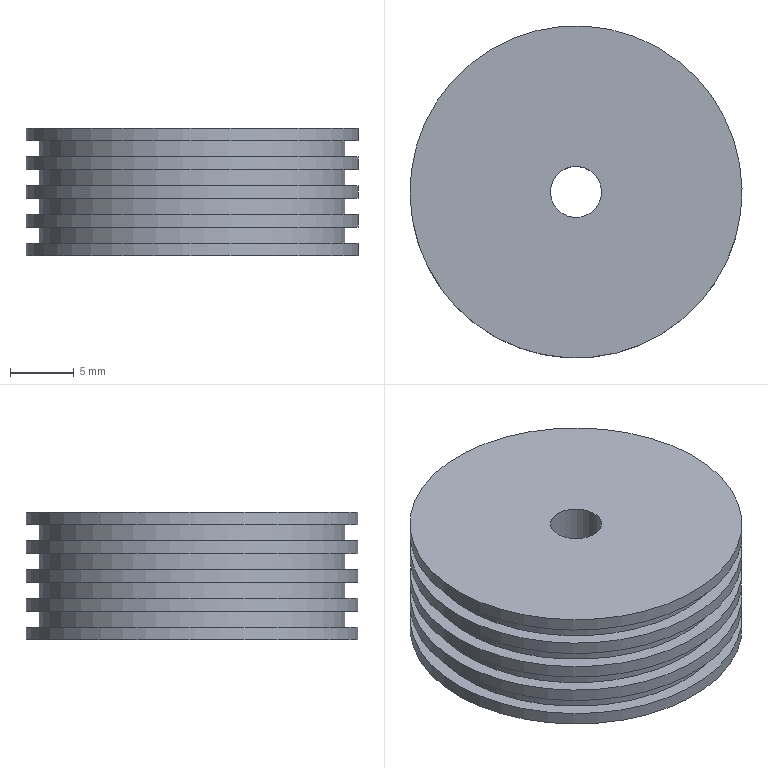Component | NX | 18A__27_2 | 1 solid | 20 faces | box 26 x 26 x 10 mm | volume 4791 mm3 | plane 10 | cylinder 10 | commonest cylinder face diameters 26 x5 24 x4 4 x1
STEP:
#1=CARTESIAN_POINT('',(0.,0.,0.));
#2=DIRECTION('',(0.,0.,1.));
#3=DIRECTION('',(1.,0.,0.));
#4=AXIS2_PLACEMENT_3D('',#1,#2,#3);
#5=CARTESIAN_POINT('',(16.256,111.456,213.535));
#6=VERTEX_POINT('',#5);
#7=CARTESIAN_POINT('',(17.022,109.608,213.535));
#8=DIRECTION('',(0.,0.,1.));
#9=DIRECTION('',(-0.383,0.9237,0.));
#10=AXIS2_PLACEMENT_3D('',#7,#8,#9);
#11=CIRCLE('',#10,2.);
#12=CARTESIAN_POINT('',(22.002,97.6,213.535));
#13=DIRECTION('',(0.,0.,-1.));
#14=DIRECTION('',(0.383,-0.9237,0.));
#15=AXIS2_PLACEMENT_3D('',#12,#13,#14);
#16=PLANE('',#15);
#17=CARTESIAN_POINT('',(-15.,0.));
#18=CARTESIAN_POINT('',(-15.,3.464));
#19=CARTESIAN_POINT('',(-12.,1.732));
#20=CARTESIAN_POINT('',(-9.,0.));
#21=CARTESIAN_POINT('',(-12.,-1.732));
#22=CARTESIAN_POINT('',(-15.,-3.464));
#23=CARTESIAN_POINT('',(-15.,0.));
#24=(BOUNDED_CURVE()B_SPLINE_CURVE(2,(#17,#18,#19,#20,#21,#22,#23),.UNSPECIFIED.,.T.,.F.)B_SPLINE_CURVE_WITH_KNOTS((1,2,2,2,2,1),(-2.094,0.,2.094,4.189,6.283,8.378),.UNSPECIFIED.)CURVE()GEOMETRIC_REPRESENTATION_ITEM()RATIONAL_B_SPLINE_CURVE((1.,0.5,1.,0.5,1.,0.5,1.))REPRESENTATION_ITEM(''));
#25=(GEOMETRIC_REPRESENTATION_CONTEXT(2)PARAMETRIC_REPRESENTATION_CONTEXT()REPRESENTATION_CONTEXT('',''));
#26=DEFINITIONAL_REPRESENTATION('',(#24),#25);
#27=PCURVE('',#16,#26);
#28=CARTESIAN_POINT('',(17.022,109.608,213.535));
#29=DIRECTION('',(0.,0.,1.));
#30=DIRECTION('',(-0.383,0.9237,0.));
#31=AXIS2_PLACEMENT_3D('',#28,#29,#30);
#32=CYLINDRICAL_SURFACE('',#31,2.);
#33=CARTESIAN_POINT('',(0.,0.));
#34=DIRECTION('',(1.,0.));
#35=VECTOR('',#34,1.);
#36=LINE('',#33,#35);
#37=(GEOMETRIC_REPRESENTATION_CONTEXT(2)PARAMETRIC_REPRESENTATION_CONTEXT()REPRESENTATION_CONTEXT('',''));
#38=DEFINITIONAL_REPRESENTATION('',(#36),#37);
#39=PCURVE('',#32,#38);
#40=SURFACE_CURVE('',#11,(#27,#39),.PCURVE_S1.);
#41=EDGE_CURVE('',#6,#6,#40,.T.);
#42=ORIENTED_EDGE('',*,*,#41,.T.);
#43=EDGE_LOOP('',(#42));
#44=FACE_BOUND('',#43,.T.);
#45=CARTESIAN_POINT('',(12.043,121.617,213.535));
#46=VERTEX_POINT('',#45);
#47=CARTESIAN_POINT('',(17.022,109.608,213.535));
#48=DIRECTION('',(0.,0.,1.));
#49=DIRECTION('',(-0.383,0.9237,0.));
#50=AXIS2_PLACEMENT_3D('',#47,#48,#49);
#51=CIRCLE('',#50,13.);
#52=CARTESIAN_POINT('',(-26.,0.));
#53=CARTESIAN_POINT('',(-26.,22.517));
#54=CARTESIAN_POINT('',(-6.5,11.258));
#55=CARTESIAN_POINT('',(13.,0.));
#56=CARTESIAN_POINT('',(-6.5,-11.258));
#57=CARTESIAN_POINT('',(-26.,-22.517));
#58=CARTESIAN_POINT('',(-26.,0.));
#59=(BOUNDED_CURVE()B_SPLINE_CURVE(2,(#52,#53,#54,#55,#56,#57,#58),.UNSPECIFIED.,.T.,.F.)B_SPLINE_CURVE_WITH_KNOTS((1,2,2,2,2,1),(-2.094,0.,2.094,4.189,6.283,8.378),.UNSPECIFIED.)CURVE()GEOMETRIC_REPRESENTATION_ITEM()RATIONAL_B_SPLINE_CURVE((1.,0.5,1.,0.5,1.,0.5,1.))REPRESENTATION_ITEM(''));
#60=(GEOMETRIC_REPRESENTATION_CONTEXT(2)PARAMETRIC_REPRESENTATION_CONTEXT()REPRESENTATION_CONTEXT('',''));
#61=DEFINITIONAL_REPRESENTATION('',(#59),#60);
#62=PCURVE('',#16,#61);
#63=CARTESIAN_POINT('',(17.022,109.608,213.535));
#64=DIRECTION('',(0.,0.,1.));
#65=DIRECTION('',(-0.383,0.9237,0.));
#66=AXIS2_PLACEMENT_3D('',#63,#64,#65);
#67=CYLINDRICAL_SURFACE('',#66,13.);
#68=CARTESIAN_POINT('',(0.,0.));
#69=DIRECTION('',(1.,0.));
#70=VECTOR('',#69,1.);
#71=LINE('',#68,#70);
#72=(GEOMETRIC_REPRESENTATION_CONTEXT(2)PARAMETRIC_REPRESENTATION_CONTEXT()REPRESENTATION_CONTEXT('',''));
#73=DEFINITIONAL_REPRESENTATION('',(#71),#72);
#74=PCURVE('',#67,#73);
#75=SURFACE_CURVE('',#51,(#62,#74),.PCURVE_S1.);
#76=EDGE_CURVE('',#46,#46,#75,.T.);
#77=ORIENTED_EDGE('',*,*,#76,.F.);
#78=EDGE_LOOP('',(#77));
#79=FACE_BOUND('',#78,.T.);
#80=ADVANCED_FACE('',(#44,#79),#16,.T.);
#81=CARTESIAN_POINT('',(16.256,111.456,223.535));
#82=VERTEX_POINT('',#81);
#83=CARTESIAN_POINT('',(17.022,109.608,223.535));
#84=DIRECTION('',(0.,0.,1.));
#85=DIRECTION('',(-0.383,0.9237,0.));
#86=AXIS2_PLACEMENT_3D('',#83,#84,#85);
#87=CIRCLE('',#86,2.);
#88=CARTESIAN_POINT('',(0.,10.));
#89=DIRECTION('',(1.,0.));
#90=VECTOR('',#89,1.);
#91=LINE('',#88,#90);
#92=(GEOMETRIC_REPRESENTATION_CONTEXT(2)PARAMETRIC_REPRESENTATION_CONTEXT()REPRESENTATION_CONTEXT('',''));
#93=DEFINITIONAL_REPRESENTATION('',(#91),#92);
#94=PCURVE('',#32,#93);
#95=CARTESIAN_POINT('',(17.788,107.761,223.535));
#96=DIRECTION('',(0.,0.,1.));
#97=DIRECTION('',(-0.383,0.9237,0.));
#98=AXIS2_PLACEMENT_3D('',#95,#96,#97);
#99=PLANE('',#98);
#100=CARTESIAN_POINT('',(2.,0.));
#101=DIRECTION('',(1.,0.));
#102=AXIS2_PLACEMENT_2D('',#100,#101);
#103=CIRCLE('',#102,2.);
#104=(GEOMETRIC_REPRESENTATION_CONTEXT(2)PARAMETRIC_REPRESENTATION_CONTEXT()REPRESENTATION_CONTEXT('',''));
#105=DEFINITIONAL_REPRESENTATION('',(#103),#104);
#106=PCURVE('',#99,#105);
#107=SURFACE_CURVE('',#87,(#94,#106),.PCURVE_S1.);
#108=EDGE_CURVE('',#82,#82,#107,.T.);
#109=ORIENTED_EDGE('',*,*,#108,.F.);
#110=CARTESIAN_POINT('',(16.256,111.456,213.535));
#111=CARTESIAN_POINT('',(16.256,111.456,223.535));
#112=B_SPLINE_CURVE_WITH_KNOTS('',1,(#110,#111),.UNSPECIFIED.,.F.,.F.,(2,2),(0.,10.),.PIECEWISE_BEZIER_KNOTS.);
#113=CARTESIAN_POINT('',(0.,0.));
#114=DIRECTION('',(0.,1.));
#115=VECTOR('',#114,1.);
#116=LINE('',#113,#115);
#117=(GEOMETRIC_REPRESENTATION_CONTEXT(2)PARAMETRIC_REPRESENTATION_CONTEXT()REPRESENTATION_CONTEXT('',''));
#118=DEFINITIONAL_REPRESENTATION('',(#116),#117);
#119=PCURVE('',#32,#118);
#120=CARTESIAN_POINT('',(6.283,0.));
#121=DIRECTION('',(0.,1.));
#122=VECTOR('',#121,1.);
#123=LINE('',#120,#122);
#124=(GEOMETRIC_REPRESENTATION_CONTEXT(2)PARAMETRIC_REPRESENTATION_CONTEXT()REPRESENTATION_CONTEXT('',''));
#125=DEFINITIONAL_REPRESENTATION('',(#123),#124);
#126=PCURVE('',#32,#125);
#127=SEAM_CURVE('',#112,(#119,#126),.PCURVE_S1.);
#128=EDGE_CURVE('',#6,#82,#127,.T.);
#129=ORIENTED_EDGE('',*,*,#128,.F.);
#130=ORIENTED_EDGE('',*,*,#41,.T.);
#131=ORIENTED_EDGE('',*,*,#128,.T.);
#132=EDGE_LOOP('',(#109,#129,#130,#131));
#133=FACE_BOUND('',#132,.F.);
#134=ADVANCED_FACE('',(#133),#32,.F.);
#135=CARTESIAN_POINT('',(12.043,121.617,223.535));
#136=VERTEX_POINT('',#135);
#137=CARTESIAN_POINT('',(17.022,109.608,223.535));
#138=DIRECTION('',(0.,0.,1.));
#139=DIRECTION('',(-0.383,0.9237,0.));
#140=AXIS2_PLACEMENT_3D('',#137,#138,#139);
#141=CIRCLE('',#140,13.);
#142=CARTESIAN_POINT('',(2.,0.));
#143=DIRECTION('',(1.,0.));
#144=AXIS2_PLACEMENT_2D('',#142,#143);
#145=CIRCLE('',#144,13.);
#146=(GEOMETRIC_REPRESENTATION_CONTEXT(2)PARAMETRIC_REPRESENTATION_CONTEXT()REPRESENTATION_CONTEXT('',''));
#147=DEFINITIONAL_REPRESENTATION('',(#145),#146);
#148=PCURVE('',#99,#147);
#149=CARTESIAN_POINT('',(17.022,109.608,213.535));
#150=DIRECTION('',(0.,0.,1.));
#151=DIRECTION('',(-0.383,0.9237,0.));
#152=AXIS2_PLACEMENT_3D('',#149,#150,#151);
#153=CYLINDRICAL_SURFACE('',#152,13.);
#154=CARTESIAN_POINT('',(0.,10.));
#155=DIRECTION('',(1.,0.));
#156=VECTOR('',#155,1.);
#157=LINE('',#154,#156);
#158=(GEOMETRIC_REPRESENTATION_CONTEXT(2)PARAMETRIC_REPRESENTATION_CONTEXT()REPRESENTATION_CONTEXT('',''));
#159=DEFINITIONAL_REPRESENTATION('',(#157),#158);
#160=PCURVE('',#153,#159);
#161=SURFACE_CURVE('',#141,(#148,#160),.PCURVE_S1.);
#162=EDGE_CURVE('',#136,#136,#161,.T.);
#163=ORIENTED_EDGE('',*,*,#162,.T.);
#164=EDGE_LOOP('',(#163));
#165=FACE_BOUND('',#164,.T.);
#166=ORIENTED_EDGE('',*,*,#108,.F.);
#167=EDGE_LOOP('',(#166));
#168=FACE_BOUND('',#167,.T.);
#169=ADVANCED_FACE('',(#165,#168),#99,.T.);
#170=CARTESIAN_POINT('',(12.043,121.617,222.535));
#171=VERTEX_POINT('',#170);
#172=CARTESIAN_POINT('',(17.022,109.608,222.535));
#173=DIRECTION('',(0.,0.,1.));
#174=DIRECTION('',(-0.383,0.9237,0.));
#175=AXIS2_PLACEMENT_3D('',#172,#173,#174);
#176=CIRCLE('',#175,13.);
#177=CARTESIAN_POINT('',(0.,9.));
#178=DIRECTION('',(1.,0.));
#179=VECTOR('',#178,1.);
#180=LINE('',#177,#179);
#181=(GEOMETRIC_REPRESENTATION_CONTEXT(2)PARAMETRIC_REPRESENTATION_CONTEXT()REPRESENTATION_CONTEXT('',''));
#182=DEFINITIONAL_REPRESENTATION('',(#180),#181);
#183=PCURVE('',#153,#182);
#184=CARTESIAN_POINT('',(22.002,97.6,222.535));
#185=DIRECTION('',(0.,0.,-1.));
#186=DIRECTION('',(0.383,-0.9237,0.));
#187=AXIS2_PLACEMENT_3D('',#184,#185,#186);
#188=PLANE('',#187);
#189=CARTESIAN_POINT('',(-26.,0.));
#190=CARTESIAN_POINT('',(-26.,22.517));
#191=CARTESIAN_POINT('',(-6.5,11.258));
#192=CARTESIAN_POINT('',(13.,0.));
#193=CARTESIAN_POINT('',(-6.5,-11.258));
#194=CARTESIAN_POINT('',(-26.,-22.517));
#195=CARTESIAN_POINT('',(-26.,0.));
#196=(BOUNDED_CURVE()B_SPLINE_CURVE(2,(#189,#190,#191,#192,#193,#194,#195),.UNSPECIFIED.,.T.,.F.)B_SPLINE_CURVE_WITH_KNOTS((1,2,2,2,2,1),(-2.094,0.,2.094,4.189,6.283,8.378),.UNSPECIFIED.)CURVE()GEOMETRIC_REPRESENTATION_ITEM()RATIONAL_B_SPLINE_CURVE((1.,0.5,1.,0.5,1.,0.5,1.))REPRESENTATION_ITEM(''));
#197=(GEOMETRIC_REPRESENTATION_CONTEXT(2)PARAMETRIC_REPRESENTATION_CONTEXT()REPRESENTATION_CONTEXT('',''));
#198=DEFINITIONAL_REPRESENTATION('',(#196),#197);
#199=PCURVE('',#188,#198);
#200=SURFACE_CURVE('',#176,(#183,#199),.PCURVE_S1.);
#201=EDGE_CURVE('',#171,#171,#200,.T.);
#202=ORIENTED_EDGE('',*,*,#201,.T.);
#203=CARTESIAN_POINT('',(12.043,121.617,222.535));
#204=CARTESIAN_POINT('',(12.043,121.617,223.535));
#205=B_SPLINE_CURVE_WITH_KNOTS('',1,(#203,#204),.UNSPECIFIED.,.F.,.F.,(2,2),(9.,10.),.PIECEWISE_BEZIER_KNOTS.);
#206=CARTESIAN_POINT('',(6.283,0.));
#207=DIRECTION('',(0.,1.));
#208=VECTOR('',#207,1.);
#209=LINE('',#206,#208);
#210=(GEOMETRIC_REPRESENTATION_CONTEXT(2)PARAMETRIC_REPRESENTATION_CONTEXT()REPRESENTATION_CONTEXT('',''));
#211=DEFINITIONAL_REPRESENTATION('',(#209),#210);
#212=PCURVE('',#153,#211);
#213=CARTESIAN_POINT('',(0.,0.));
#214=DIRECTION('',(0.,1.));
#215=VECTOR('',#214,1.);
#216=LINE('',#213,#215);
#217=(GEOMETRIC_REPRESENTATION_CONTEXT(2)PARAMETRIC_REPRESENTATION_CONTEXT()REPRESENTATION_CONTEXT('',''));
#218=DEFINITIONAL_REPRESENTATION('',(#216),#217);
#219=PCURVE('',#153,#218);
#220=SEAM_CURVE('',#205,(#212,#219),.PCURVE_S1.);
#221=EDGE_CURVE('',#171,#136,#220,.T.);
#222=ORIENTED_EDGE('',*,*,#221,.T.);
#223=ORIENTED_EDGE('',*,*,#162,.F.);
#224=ORIENTED_EDGE('',*,*,#221,.F.);
#225=EDGE_LOOP('',(#202,#222,#223,#224));
#226=FACE_BOUND('',#225,.T.);
#227=ADVANCED_FACE('',(#226),#153,.T.);
#228=CARTESIAN_POINT('',(12.426,120.693,222.535));
#229=VERTEX_POINT('',#228);
#230=CARTESIAN_POINT('',(17.022,109.608,222.535));
#231=DIRECTION('',(0.,0.,1.));
#232=DIRECTION('',(-0.383,0.9237,0.));
#233=AXIS2_PLACEMENT_3D('',#230,#231,#232);
#234=CIRCLE('',#233,12.);
#235=CARTESIAN_POINT('',(-25.,0.));
#236=CARTESIAN_POINT('',(-25.,20.785));
#237=CARTESIAN_POINT('',(-7.,10.392));
#238=CARTESIAN_POINT('',(11.,0.));
#239=CARTESIAN_POINT('',(-7.,-10.392));
#240=CARTESIAN_POINT('',(-25.,-20.785));
#241=CARTESIAN_POINT('',(-25.,0.));
#242=(BOUNDED_CURVE()B_SPLINE_CURVE(2,(#235,#236,#237,#238,#239,#240,#241),.UNSPECIFIED.,.T.,.F.)B_SPLINE_CURVE_WITH_KNOTS((1,2,2,2,2,1),(-2.094,0.,2.094,4.189,6.283,8.378),.UNSPECIFIED.)CURVE()GEOMETRIC_REPRESENTATION_ITEM()RATIONAL_B_SPLINE_CURVE((1.,0.5,1.,0.5,1.,0.5,1.))REPRESENTATION_ITEM(''));
#243=(GEOMETRIC_REPRESENTATION_CONTEXT(2)PARAMETRIC_REPRESENTATION_CONTEXT()REPRESENTATION_CONTEXT('',''));
#244=DEFINITIONAL_REPRESENTATION('',(#242),#243);
#245=PCURVE('',#188,#244);
#246=CARTESIAN_POINT('',(17.022,109.608,213.535));
#247=DIRECTION('',(0.,0.,1.));
#248=DIRECTION('',(-0.383,0.9237,0.));
#249=AXIS2_PLACEMENT_3D('',#246,#247,#248);
#250=CYLINDRICAL_SURFACE('',#249,12.);
#251=CARTESIAN_POINT('',(0.,9.));
#252=DIRECTION('',(1.,0.));
#253=VECTOR('',#252,1.);
#254=LINE('',#251,#253);
#255=(GEOMETRIC_REPRESENTATION_CONTEXT(2)PARAMETRIC_REPRESENTATION_CONTEXT()REPRESENTATION_CONTEXT('',''));
#256=DEFINITIONAL_REPRESENTATION('',(#254),#255);
#257=PCURVE('',#250,#256);
#258=SURFACE_CURVE('',#234,(#245,#257),.PCURVE_S1.);
#259=EDGE_CURVE('',#229,#229,#258,.T.);
#260=ORIENTED_EDGE('',*,*,#259,.T.);
#261=EDGE_LOOP('',(#260));
#262=FACE_BOUND('',#261,.T.);
#263=ORIENTED_EDGE('',*,*,#201,.F.);
#264=EDGE_LOOP('',(#263));
#265=FACE_BOUND('',#264,.T.);
#266=ADVANCED_FACE('',(#262,#265),#188,.T.);
#267=CARTESIAN_POINT('',(12.426,120.693,221.285));
#268=VERTEX_POINT('',#267);
#269=CARTESIAN_POINT('',(17.022,109.608,221.285));
#270=DIRECTION('',(0.,0.,1.));
#271=DIRECTION('',(-0.383,0.9237,0.));
#272=AXIS2_PLACEMENT_3D('',#269,#270,#271);
#273=CIRCLE('',#272,12.);
#274=CARTESIAN_POINT('',(0.,7.75));
#275=DIRECTION('',(1.,0.));
#276=VECTOR('',#275,1.);
#277=LINE('',#274,#276);
#278=(GEOMETRIC_REPRESENTATION_CONTEXT(2)PARAMETRIC_REPRESENTATION_CONTEXT()REPRESENTATION_CONTEXT('',''));
#279=DEFINITIONAL_REPRESENTATION('',(#277),#278);
#280=PCURVE('',#250,#279);
#281=CARTESIAN_POINT('',(21.619,98.523,221.285));
#282=DIRECTION('',(0.,0.,1.));
#283=DIRECTION('',(-0.383,0.9237,0.));
#284=AXIS2_PLACEMENT_3D('',#281,#282,#283);
#285=PLANE('',#284);
#286=CARTESIAN_POINT('',(12.,0.));
#287=DIRECTION('',(1.,0.));
#288=AXIS2_PLACEMENT_2D('',#286,#287);
#289=CIRCLE('',#288,12.);
#290=(GEOMETRIC_REPRESENTATION_CONTEXT(2)PARAMETRIC_REPRESENTATION_CONTEXT()REPRESENTATION_CONTEXT('',''));
#291=DEFINITIONAL_REPRESENTATION('',(#289),#290);
#292=PCURVE('',#285,#291);
#293=SURFACE_CURVE('',#273,(#280,#292),.PCURVE_S1.);
#294=EDGE_CURVE('',#268,#268,#293,.T.);
#295=ORIENTED_EDGE('',*,*,#294,.T.);
#296=CARTESIAN_POINT('',(12.426,120.693,221.285));
#297=CARTESIAN_POINT('',(12.426,120.693,222.535));
#298=B_SPLINE_CURVE_WITH_KNOTS('',1,(#296,#297),.UNSPECIFIED.,.F.,.F.,(2,2),(7.75,9.),.PIECEWISE_BEZIER_KNOTS.);
#299=CARTESIAN_POINT('',(6.283,0.));
#300=DIRECTION('',(0.,1.));
#301=VECTOR('',#300,1.);
#302=LINE('',#299,#301);
#303=(GEOMETRIC_REPRESENTATION_CONTEXT(2)PARAMETRIC_REPRESENTATION_CONTEXT()REPRESENTATION_CONTEXT('',''));
#304=DEFINITIONAL_REPRESENTATION('',(#302),#303);
#305=PCURVE('',#250,#304);
#306=CARTESIAN_POINT('',(0.,0.));
#307=DIRECTION('',(0.,1.));
#308=VECTOR('',#307,1.);
#309=LINE('',#306,#308);
#310=(GEOMETRIC_REPRESENTATION_CONTEXT(2)PARAMETRIC_REPRESENTATION_CONTEXT()REPRESENTATION_CONTEXT('',''));
#311=DEFINITIONAL_REPRESENTATION('',(#309),#310);
#312=PCURVE('',#250,#311);
#313=SEAM_CURVE('',#298,(#305,#312),.PCURVE_S1.);
#314=EDGE_CURVE('',#268,#229,#313,.T.);
#315=ORIENTED_EDGE('',*,*,#314,.T.);
#316=ORIENTED_EDGE('',*,*,#259,.F.);
#317=ORIENTED_EDGE('',*,*,#314,.F.);
#318=EDGE_LOOP('',(#295,#315,#316,#317));
#319=FACE_BOUND('',#318,.T.);
#320=ADVANCED_FACE('',(#319),#250,.T.);
#321=CARTESIAN_POINT('',(12.043,121.617,221.285));
#322=VERTEX_POINT('',#321);
#323=CARTESIAN_POINT('',(17.022,109.608,221.285));
#324=DIRECTION('',(0.,0.,1.));
#325=DIRECTION('',(-0.383,0.9237,0.));
#326=AXIS2_PLACEMENT_3D('',#323,#324,#325);
#327=CIRCLE('',#326,13.);
#328=CARTESIAN_POINT('',(12.,0.));
#329=DIRECTION('',(1.,0.));
#330=AXIS2_PLACEMENT_2D('',#328,#329);
#331=CIRCLE('',#330,13.);
#332=(GEOMETRIC_REPRESENTATION_CONTEXT(2)PARAMETRIC_REPRESENTATION_CONTEXT()REPRESENTATION_CONTEXT('',''));
#333=DEFINITIONAL_REPRESENTATION('',(#331),#332);
#334=PCURVE('',#285,#333);
#335=CARTESIAN_POINT('',(17.022,109.608,213.535));
#336=DIRECTION('',(0.,0.,1.));
#337=DIRECTION('',(-0.383,0.9237,0.));
#338=AXIS2_PLACEMENT_3D('',#335,#336,#337);
#339=CYLINDRICAL_SURFACE('',#338,13.);
#340=CARTESIAN_POINT('',(0.,7.75));
#341=DIRECTION('',(1.,0.));
#342=VECTOR('',#341,1.);
#343=LINE('',#340,#342);
#344=(GEOMETRIC_REPRESENTATION_CONTEXT(2)PARAMETRIC_REPRESENTATION_CONTEXT()REPRESENTATION_CONTEXT('',''));
#345=DEFINITIONAL_REPRESENTATION('',(#343),#344);
#346=PCURVE('',#339,#345);
#347=SURFACE_CURVE('',#327,(#334,#346),.PCURVE_S1.);
#348=EDGE_CURVE('',#322,#322,#347,.T.);
#349=ORIENTED_EDGE('',*,*,#348,.T.);
#350=EDGE_LOOP('',(#349));
#351=FACE_BOUND('',#350,.T.);
#352=ORIENTED_EDGE('',*,*,#294,.F.);
#353=EDGE_LOOP('',(#352));
#354=FACE_BOUND('',#353,.T.);
#355=ADVANCED_FACE('',(#351,#354),#285,.T.);
#356=CARTESIAN_POINT('',(12.043,121.617,220.285));
#357=VERTEX_POINT('',#356);
#358=CARTESIAN_POINT('',(17.022,109.608,220.285));
#359=DIRECTION('',(0.,0.,1.));
#360=DIRECTION('',(-0.383,0.9237,0.));
#361=AXIS2_PLACEMENT_3D('',#358,#359,#360);
#362=CIRCLE('',#361,13.);
#363=CARTESIAN_POINT('',(0.,6.75));
#364=DIRECTION('',(1.,0.));
#365=VECTOR('',#364,1.);
#366=LINE('',#363,#365);
#367=(GEOMETRIC_REPRESENTATION_CONTEXT(2)PARAMETRIC_REPRESENTATION_CONTEXT()REPRESENTATION_CONTEXT('',''));
#368=DEFINITIONAL_REPRESENTATION('',(#366),#367);
#369=PCURVE('',#339,#368);
#370=CARTESIAN_POINT('',(22.002,97.6,220.285));
#371=DIRECTION('',(0.,0.,-1.));
#372=DIRECTION('',(0.383,-0.9237,0.));
#373=AXIS2_PLACEMENT_3D('',#370,#371,#372);
#374=PLANE('',#373);
#375=CARTESIAN_POINT('',(-26.,0.));
#376=CARTESIAN_POINT('',(-26.,22.517));
#377=CARTESIAN_POINT('',(-6.5,11.258));
#378=CARTESIAN_POINT('',(13.,0.));
#379=CARTESIAN_POINT('',(-6.5,-11.258));
#380=CARTESIAN_POINT('',(-26.,-22.517));
#381=CARTESIAN_POINT('',(-26.,0.));
#382=(BOUNDED_CURVE()B_SPLINE_CURVE(2,(#375,#376,#377,#378,#379,#380,#381),.UNSPECIFIED.,.T.,.F.)B_SPLINE_CURVE_WITH_KNOTS((1,2,2,2,2,1),(-2.094,0.,2.094,4.189,6.283,8.378),.UNSPECIFIED.)CURVE()GEOMETRIC_REPRESENTATION_ITEM()RATIONAL_B_SPLINE_CURVE((1.,0.5,1.,0.5,1.,0.5,1.))REPRESENTATION_ITEM(''));
#383=(GEOMETRIC_REPRESENTATION_CONTEXT(2)PARAMETRIC_REPRESENTATION_CONTEXT()REPRESENTATION_CONTEXT('',''));
#384=DEFINITIONAL_REPRESENTATION('',(#382),#383);
#385=PCURVE('',#374,#384);
#386=SURFACE_CURVE('',#362,(#369,#385),.PCURVE_S1.);
#387=EDGE_CURVE('',#357,#357,#386,.T.);
#388=ORIENTED_EDGE('',*,*,#387,.T.);
#389=CARTESIAN_POINT('',(12.043,121.617,220.285));
#390=CARTESIAN_POINT('',(12.043,121.617,221.285));
#391=B_SPLINE_CURVE_WITH_KNOTS('',1,(#389,#390),.UNSPECIFIED.,.F.,.F.,(2,2),(6.75,7.75),.PIECEWISE_BEZIER_KNOTS.);
#392=CARTESIAN_POINT('',(6.283,0.));
#393=DIRECTION('',(0.,1.));
#394=VECTOR('',#393,1.);
#395=LINE('',#392,#394);
#396=(GEOMETRIC_REPRESENTATION_CONTEXT(2)PARAMETRIC_REPRESENTATION_CONTEXT()REPRESENTATION_CONTEXT('',''));
#397=DEFINITIONAL_REPRESENTATION('',(#395),#396);
#398=PCURVE('',#339,#397);
#399=CARTESIAN_POINT('',(0.,0.));
#400=DIRECTION('',(0.,1.));
#401=VECTOR('',#400,1.);
#402=LINE('',#399,#401);
#403=(GEOMETRIC_REPRESENTATION_CONTEXT(2)PARAMETRIC_REPRESENTATION_CONTEXT()REPRESENTATION_CONTEXT('',''));
#404=DEFINITIONAL_REPRESENTATION('',(#402),#403);
#405=PCURVE('',#339,#404);
#406=SEAM_CURVE('',#391,(#398,#405),.PCURVE_S1.);
#407=EDGE_CURVE('',#357,#322,#406,.T.);
#408=ORIENTED_EDGE('',*,*,#407,.T.);
#409=ORIENTED_EDGE('',*,*,#348,.F.);
#410=ORIENTED_EDGE('',*,*,#407,.F.);
#411=EDGE_LOOP('',(#388,#408,#409,#410));
#412=FACE_BOUND('',#411,.T.);
#413=ADVANCED_FACE('',(#412),#339,.T.);
#414=CARTESIAN_POINT('',(12.426,120.693,220.285));
#415=VERTEX_POINT('',#414);
#416=CARTESIAN_POINT('',(17.022,109.608,220.285));
#417=DIRECTION('',(0.,0.,1.));
#418=DIRECTION('',(-0.383,0.9237,0.));
#419=AXIS2_PLACEMENT_3D('',#416,#417,#418);
#420=CIRCLE('',#419,12.);
#421=CARTESIAN_POINT('',(-25.,0.));
#422=CARTESIAN_POINT('',(-25.,20.785));
#423=CARTESIAN_POINT('',(-7.,10.392));
#424=CARTESIAN_POINT('',(11.,0.));
#425=CARTESIAN_POINT('',(-7.,-10.392));
#426=CARTESIAN_POINT('',(-25.,-20.785));
#427=CARTESIAN_POINT('',(-25.,0.));
#428=(BOUNDED_CURVE()B_SPLINE_CURVE(2,(#421,#422,#423,#424,#425,#426,#427),.UNSPECIFIED.,.T.,.F.)B_SPLINE_CURVE_WITH_KNOTS((1,2,2,2,2,1),(-2.094,0.,2.094,4.189,6.283,8.378),.UNSPECIFIED.)CURVE()GEOMETRIC_REPRESENTATION_ITEM()RATIONAL_B_SPLINE_CURVE((1.,0.5,1.,0.5,1.,0.5,1.))REPRESENTATION_ITEM(''));
#429=(GEOMETRIC_REPRESENTATION_CONTEXT(2)PARAMETRIC_REPRESENTATION_CONTEXT()REPRESENTATION_CONTEXT('',''));
#430=DEFINITIONAL_REPRESENTATION('',(#428),#429);
#431=PCURVE('',#374,#430);
#432=CARTESIAN_POINT('',(17.022,109.608,213.535));
#433=DIRECTION('',(0.,0.,1.));
#434=DIRECTION('',(-0.383,0.9237,0.));
#435=AXIS2_PLACEMENT_3D('',#432,#433,#434);
#436=CYLINDRICAL_SURFACE('',#435,12.);
#437=CARTESIAN_POINT('',(0.,6.75));
#438=DIRECTION('',(1.,0.));
#439=VECTOR('',#438,1.);
#440=LINE('',#437,#439);
#441=(GEOMETRIC_REPRESENTATION_CONTEXT(2)PARAMETRIC_REPRESENTATION_CONTEXT()REPRESENTATION_CONTEXT('',''));
#442=DEFINITIONAL_REPRESENTATION('',(#440),#441);
#443=PCURVE('',#436,#442);
#444=SURFACE_CURVE('',#420,(#431,#443),.PCURVE_S1.);
#445=EDGE_CURVE('',#415,#415,#444,.T.);
#446=ORIENTED_EDGE('',*,*,#445,.T.);
#447=EDGE_LOOP('',(#446));
#448=FACE_BOUND('',#447,.T.);
#449=ORIENTED_EDGE('',*,*,#387,.F.);
#450=EDGE_LOOP('',(#449));
#451=FACE_BOUND('',#450,.T.);
#452=ADVANCED_FACE('',(#448,#451),#374,.T.);
#453=CARTESIAN_POINT('',(12.426,120.693,219.035));
#454=VERTEX_POINT('',#453);
#455=CARTESIAN_POINT('',(17.022,109.608,219.035));
#456=DIRECTION('',(0.,0.,1.));
#457=DIRECTION('',(-0.383,0.9237,0.));
#458=AXIS2_PLACEMENT_3D('',#455,#456,#457);
#459=CIRCLE('',#458,12.);
#460=CARTESIAN_POINT('',(0.,5.5));
#461=DIRECTION('',(1.,0.));
#462=VECTOR('',#461,1.);
#463=LINE('',#460,#462);
#464=(GEOMETRIC_REPRESENTATION_CONTEXT(2)PARAMETRIC_REPRESENTATION_CONTEXT()REPRESENTATION_CONTEXT('',''));
#465=DEFINITIONAL_REPRESENTATION('',(#463),#464);
#466=PCURVE('',#436,#465);
#467=CARTESIAN_POINT('',(21.619,98.523,219.035));
#468=DIRECTION('',(0.,0.,1.));
#469=DIRECTION('',(-0.383,0.9237,0.));
#470=AXIS2_PLACEMENT_3D('',#467,#468,#469);
#471=PLANE('',#470);
#472=CARTESIAN_POINT('',(12.,0.));
#473=DIRECTION('',(1.,0.));
#474=AXIS2_PLACEMENT_2D('',#472,#473);
#475=CIRCLE('',#474,12.);
#476=(GEOMETRIC_REPRESENTATION_CONTEXT(2)PARAMETRIC_REPRESENTATION_CONTEXT()REPRESENTATION_CONTEXT('',''));
#477=DEFINITIONAL_REPRESENTATION('',(#475),#476);
#478=PCURVE('',#471,#477);
#479=SURFACE_CURVE('',#459,(#466,#478),.PCURVE_S1.);
#480=EDGE_CURVE('',#454,#454,#479,.T.);
#481=ORIENTED_EDGE('',*,*,#480,.T.);
#482=CARTESIAN_POINT('',(12.426,120.693,219.035));
#483=CARTESIAN_POINT('',(12.426,120.693,220.285));
#484=B_SPLINE_CURVE_WITH_KNOTS('',1,(#482,#483),.UNSPECIFIED.,.F.,.F.,(2,2),(5.5,6.75),.PIECEWISE_BEZIER_KNOTS.);
#485=CARTESIAN_POINT('',(6.283,0.));
#486=DIRECTION('',(0.,1.));
#487=VECTOR('',#486,1.);
#488=LINE('',#485,#487);
#489=(GEOMETRIC_REPRESENTATION_CONTEXT(2)PARAMETRIC_REPRESENTATION_CONTEXT()REPRESENTATION_CONTEXT('',''));
#490=DEFINITIONAL_REPRESENTATION('',(#488),#489);
#491=PCURVE('',#436,#490);
#492=CARTESIAN_POINT('',(0.,0.));
#493=DIRECTION('',(0.,1.));
#494=VECTOR('',#493,1.);
#495=LINE('',#492,#494);
#496=(GEOMETRIC_REPRESENTATION_CONTEXT(2)PARAMETRIC_REPRESENTATION_CONTEXT()REPRESENTATION_CONTEXT('',''));
#497=DEFINITIONAL_REPRESENTATION('',(#495),#496);
#498=PCURVE('',#436,#497);
#499=SEAM_CURVE('',#484,(#491,#498),.PCURVE_S1.);
#500=EDGE_CURVE('',#454,#415,#499,.T.);
#501=ORIENTED_EDGE('',*,*,#500,.T.);
#502=ORIENTED_EDGE('',*,*,#445,.F.);
#503=ORIENTED_EDGE('',*,*,#500,.F.);
#504=EDGE_LOOP('',(#481,#501,#502,#503));
#505=FACE_BOUND('',#504,.T.);
#506=ADVANCED_FACE('',(#505),#436,.T.);
#507=CARTESIAN_POINT('',(12.043,121.617,219.035));
#508=VERTEX_POINT('',#507);
#509=CARTESIAN_POINT('',(17.022,109.608,219.035));
#510=DIRECTION('',(0.,0.,1.));
#511=DIRECTION('',(-0.383,0.9237,0.));
#512=AXIS2_PLACEMENT_3D('',#509,#510,#511);
#513=CIRCLE('',#512,13.);
#514=CARTESIAN_POINT('',(12.,0.));
#515=DIRECTION('',(1.,0.));
#516=AXIS2_PLACEMENT_2D('',#514,#515);
#517=CIRCLE('',#516,13.);
#518=(GEOMETRIC_REPRESENTATION_CONTEXT(2)PARAMETRIC_REPRESENTATION_CONTEXT()REPRESENTATION_CONTEXT('',''));
#519=DEFINITIONAL_REPRESENTATION('',(#517),#518);
#520=PCURVE('',#471,#519);
#521=CARTESIAN_POINT('',(17.022,109.608,213.535));
#522=DIRECTION('',(0.,0.,1.));
#523=DIRECTION('',(-0.383,0.9237,0.));
#524=AXIS2_PLACEMENT_3D('',#521,#522,#523);
#525=CYLINDRICAL_SURFACE('',#524,13.);
#526=CARTESIAN_POINT('',(0.,5.5));
#527=DIRECTION('',(1.,0.));
#528=VECTOR('',#527,1.);
#529=LINE('',#526,#528);
#530=(GEOMETRIC_REPRESENTATION_CONTEXT(2)PARAMETRIC_REPRESENTATION_CONTEXT()REPRESENTATION_CONTEXT('',''));
#531=DEFINITIONAL_REPRESENTATION('',(#529),#530);
#532=PCURVE('',#525,#531);
#533=SURFACE_CURVE('',#513,(#520,#532),.PCURVE_S1.);
#534=EDGE_CURVE('',#508,#508,#533,.T.);
#535=ORIENTED_EDGE('',*,*,#534,.T.);
#536=EDGE_LOOP('',(#535));
#537=FACE_BOUND('',#536,.T.);
#538=ORIENTED_EDGE('',*,*,#480,.F.);
#539=EDGE_LOOP('',(#538));
#540=FACE_BOUND('',#539,.T.);
#541=ADVANCED_FACE('',(#537,#540),#471,.T.);
#542=CARTESIAN_POINT('',(12.043,121.617,218.035));
#543=VERTEX_POINT('',#542);
#544=CARTESIAN_POINT('',(17.022,109.608,218.035));
#545=DIRECTION('',(0.,0.,1.));
#546=DIRECTION('',(-0.383,0.9237,0.));
#547=AXIS2_PLACEMENT_3D('',#544,#545,#546);
#548=CIRCLE('',#547,13.);
#549=CARTESIAN_POINT('',(0.,4.5));
#550=DIRECTION('',(1.,0.));
#551=VECTOR('',#550,1.);
#552=LINE('',#549,#551);
#553=(GEOMETRIC_REPRESENTATION_CONTEXT(2)PARAMETRIC_REPRESENTATION_CONTEXT()REPRESENTATION_CONTEXT('',''));
#554=DEFINITIONAL_REPRESENTATION('',(#552),#553);
#555=PCURVE('',#525,#554);
#556=CARTESIAN_POINT('',(22.002,97.6,218.035));
#557=DIRECTION('',(0.,0.,-1.));
#558=DIRECTION('',(0.383,-0.9237,0.));
#559=AXIS2_PLACEMENT_3D('',#556,#557,#558);
#560=PLANE('',#559);
#561=CARTESIAN_POINT('',(-26.,0.));
#562=CARTESIAN_POINT('',(-26.,22.517));
#563=CARTESIAN_POINT('',(-6.5,11.258));
#564=CARTESIAN_POINT('',(13.,0.));
#565=CARTESIAN_POINT('',(-6.5,-11.258));
#566=CARTESIAN_POINT('',(-26.,-22.517));
#567=CARTESIAN_POINT('',(-26.,0.));
#568=(BOUNDED_CURVE()B_SPLINE_CURVE(2,(#561,#562,#563,#564,#565,#566,#567),.UNSPECIFIED.,.T.,.F.)B_SPLINE_CURVE_WITH_KNOTS((1,2,2,2,2,1),(-2.094,0.,2.094,4.189,6.283,8.378),.UNSPECIFIED.)CURVE()GEOMETRIC_REPRESENTATION_ITEM()RATIONAL_B_SPLINE_CURVE((1.,0.5,1.,0.5,1.,0.5,1.))REPRESENTATION_ITEM(''));
#569=(GEOMETRIC_REPRESENTATION_CONTEXT(2)PARAMETRIC_REPRESENTATION_CONTEXT()REPRESENTATION_CONTEXT('',''));
#570=DEFINITIONAL_REPRESENTATION('',(#568),#569);
#571=PCURVE('',#560,#570);
#572=SURFACE_CURVE('',#548,(#555,#571),.PCURVE_S1.);
#573=EDGE_CURVE('',#543,#543,#572,.T.);
#574=ORIENTED_EDGE('',*,*,#573,.T.);
#575=CARTESIAN_POINT('',(12.043,121.617,218.035));
#576=CARTESIAN_POINT('',(12.043,121.617,219.035));
#577=B_SPLINE_CURVE_WITH_KNOTS('',1,(#575,#576),.UNSPECIFIED.,.F.,.F.,(2,2),(4.5,5.5),.PIECEWISE_BEZIER_KNOTS.);
#578=CARTESIAN_POINT('',(6.283,0.));
#579=DIRECTION('',(0.,1.));
#580=VECTOR('',#579,1.);
#581=LINE('',#578,#580);
#582=(GEOMETRIC_REPRESENTATION_CONTEXT(2)PARAMETRIC_REPRESENTATION_CONTEXT()REPRESENTATION_CONTEXT('',''));
#583=DEFINITIONAL_REPRESENTATION('',(#581),#582);
#584=PCURVE('',#525,#583);
#585=CARTESIAN_POINT('',(0.,0.));
#586=DIRECTION('',(0.,1.));
#587=VECTOR('',#586,1.);
#588=LINE('',#585,#587);
#589=(GEOMETRIC_REPRESENTATION_CONTEXT(2)PARAMETRIC_REPRESENTATION_CONTEXT()REPRESENTATION_CONTEXT('',''));
#590=DEFINITIONAL_REPRESENTATION('',(#588),#589);
#591=PCURVE('',#525,#590);
#592=SEAM_CURVE('',#577,(#584,#591),.PCURVE_S1.);
#593=EDGE_CURVE('',#543,#508,#592,.T.);
#594=ORIENTED_EDGE('',*,*,#593,.T.);
#595=ORIENTED_EDGE('',*,*,#534,.F.);
#596=ORIENTED_EDGE('',*,*,#593,.F.);
#597=EDGE_LOOP('',(#574,#594,#595,#596));
#598=FACE_BOUND('',#597,.T.);
#599=ADVANCED_FACE('',(#598),#525,.T.);
#600=CARTESIAN_POINT('',(12.426,120.693,218.035));
#601=VERTEX_POINT('',#600);
#602=CARTESIAN_POINT('',(17.022,109.608,218.035));
#603=DIRECTION('',(0.,0.,1.));
#604=DIRECTION('',(-0.383,0.9237,0.));
#605=AXIS2_PLACEMENT_3D('',#602,#603,#604);
#606=CIRCLE('',#605,12.);
#607=CARTESIAN_POINT('',(-25.,0.));
#608=CARTESIAN_POINT('',(-25.,20.785));
#609=CARTESIAN_POINT('',(-7.,10.392));
#610=CARTESIAN_POINT('',(11.,0.));
#611=CARTESIAN_POINT('',(-7.,-10.392));
#612=CARTESIAN_POINT('',(-25.,-20.785));
#613=CARTESIAN_POINT('',(-25.,0.));
#614=(BOUNDED_CURVE()B_SPLINE_CURVE(2,(#607,#608,#609,#610,#611,#612,#613),.UNSPECIFIED.,.T.,.F.)B_SPLINE_CURVE_WITH_KNOTS((1,2,2,2,2,1),(-2.094,0.,2.094,4.189,6.283,8.378),.UNSPECIFIED.)CURVE()GEOMETRIC_REPRESENTATION_ITEM()RATIONAL_B_SPLINE_CURVE((1.,0.5,1.,0.5,1.,0.5,1.))REPRESENTATION_ITEM(''));
#615=(GEOMETRIC_REPRESENTATION_CONTEXT(2)PARAMETRIC_REPRESENTATION_CONTEXT()REPRESENTATION_CONTEXT('',''));
#616=DEFINITIONAL_REPRESENTATION('',(#614),#615);
#617=PCURVE('',#560,#616);
#618=CARTESIAN_POINT('',(17.022,109.608,213.535));
#619=DIRECTION('',(0.,0.,1.));
#620=DIRECTION('',(-0.383,0.9237,0.));
#621=AXIS2_PLACEMENT_3D('',#618,#619,#620);
#622=CYLINDRICAL_SURFACE('',#621,12.);
#623=CARTESIAN_POINT('',(0.,4.5));
#624=DIRECTION('',(1.,0.));
#625=VECTOR('',#624,1.);
#626=LINE('',#623,#625);
#627=(GEOMETRIC_REPRESENTATION_CONTEXT(2)PARAMETRIC_REPRESENTATION_CONTEXT()REPRESENTATION_CONTEXT('',''));
#628=DEFINITIONAL_REPRESENTATION('',(#626),#627);
#629=PCURVE('',#622,#628);
#630=SURFACE_CURVE('',#606,(#617,#629),.PCURVE_S1.);
#631=EDGE_CURVE('',#601,#601,#630,.T.);
#632=ORIENTED_EDGE('',*,*,#631,.T.);
#633=EDGE_LOOP('',(#632));
#634=FACE_BOUND('',#633,.T.);
#635=ORIENTED_EDGE('',*,*,#573,.F.);
#636=EDGE_LOOP('',(#635));
#637=FACE_BOUND('',#636,.T.);
#638=ADVANCED_FACE('',(#634,#637),#560,.T.);
#639=CARTESIAN_POINT('',(12.426,120.693,216.785));
#640=VERTEX_POINT('',#639);
#641=CARTESIAN_POINT('',(17.022,109.608,216.785));
#642=DIRECTION('',(0.,0.,1.));
#643=DIRECTION('',(-0.383,0.9237,0.));
#644=AXIS2_PLACEMENT_3D('',#641,#642,#643);
#645=CIRCLE('',#644,12.);
#646=CARTESIAN_POINT('',(0.,3.25));
#647=DIRECTION('',(1.,0.));
#648=VECTOR('',#647,1.);
#649=LINE('',#646,#648);
#650=(GEOMETRIC_REPRESENTATION_CONTEXT(2)PARAMETRIC_REPRESENTATION_CONTEXT()REPRESENTATION_CONTEXT('',''));
#651=DEFINITIONAL_REPRESENTATION('',(#649),#650);
#652=PCURVE('',#622,#651);
#653=CARTESIAN_POINT('',(21.619,98.523,216.785));
#654=DIRECTION('',(0.,0.,1.));
#655=DIRECTION('',(-0.383,0.9237,0.));
#656=AXIS2_PLACEMENT_3D('',#653,#654,#655);
#657=PLANE('',#656);
#658=CARTESIAN_POINT('',(12.,0.));
#659=DIRECTION('',(1.,0.));
#660=AXIS2_PLACEMENT_2D('',#658,#659);
#661=CIRCLE('',#660,12.);
#662=(GEOMETRIC_REPRESENTATION_CONTEXT(2)PARAMETRIC_REPRESENTATION_CONTEXT()REPRESENTATION_CONTEXT('',''));
#663=DEFINITIONAL_REPRESENTATION('',(#661),#662);
#664=PCURVE('',#657,#663);
#665=SURFACE_CURVE('',#645,(#652,#664),.PCURVE_S1.);
#666=EDGE_CURVE('',#640,#640,#665,.T.);
#667=ORIENTED_EDGE('',*,*,#666,.T.);
#668=CARTESIAN_POINT('',(12.426,120.693,216.785));
#669=CARTESIAN_POINT('',(12.426,120.693,218.035));
#670=B_SPLINE_CURVE_WITH_KNOTS('',1,(#668,#669),.UNSPECIFIED.,.F.,.F.,(2,2),(3.25,4.5),.PIECEWISE_BEZIER_KNOTS.);
#671=CARTESIAN_POINT('',(6.283,0.));
#672=DIRECTION('',(0.,1.));
#673=VECTOR('',#672,1.);
#674=LINE('',#671,#673);
#675=(GEOMETRIC_REPRESENTATION_CONTEXT(2)PARAMETRIC_REPRESENTATION_CONTEXT()REPRESENTATION_CONTEXT('',''));
#676=DEFINITIONAL_REPRESENTATION('',(#674),#675);
#677=PCURVE('',#622,#676);
#678=CARTESIAN_POINT('',(0.,0.));
#679=DIRECTION('',(0.,1.));
#680=VECTOR('',#679,1.);
#681=LINE('',#678,#680);
#682=(GEOMETRIC_REPRESENTATION_CONTEXT(2)PARAMETRIC_REPRESENTATION_CONTEXT()REPRESENTATION_CONTEXT('',''));
#683=DEFINITIONAL_REPRESENTATION('',(#681),#682);
#684=PCURVE('',#622,#683);
#685=SEAM_CURVE('',#670,(#677,#684),.PCURVE_S1.);
#686=EDGE_CURVE('',#640,#601,#685,.T.);
#687=ORIENTED_EDGE('',*,*,#686,.T.);
#688=ORIENTED_EDGE('',*,*,#631,.F.);
#689=ORIENTED_EDGE('',*,*,#686,.F.);
#690=EDGE_LOOP('',(#667,#687,#688,#689));
#691=FACE_BOUND('',#690,.T.);
#692=ADVANCED_FACE('',(#691),#622,.T.);
#693=CARTESIAN_POINT('',(12.043,121.617,216.785));
#694=VERTEX_POINT('',#693);
#695=CARTESIAN_POINT('',(17.022,109.608,216.785));
#696=DIRECTION('',(0.,0.,1.));
#697=DIRECTION('',(-0.383,0.9237,0.));
#698=AXIS2_PLACEMENT_3D('',#695,#696,#697);
#699=CIRCLE('',#698,13.);
#700=CARTESIAN_POINT('',(12.,0.));
#701=DIRECTION('',(1.,0.));
#702=AXIS2_PLACEMENT_2D('',#700,#701);
#703=CIRCLE('',#702,13.);
#704=(GEOMETRIC_REPRESENTATION_CONTEXT(2)PARAMETRIC_REPRESENTATION_CONTEXT()REPRESENTATION_CONTEXT('',''));
#705=DEFINITIONAL_REPRESENTATION('',(#703),#704);
#706=PCURVE('',#657,#705);
#707=CARTESIAN_POINT('',(17.022,109.608,213.535));
#708=DIRECTION('',(0.,0.,1.));
#709=DIRECTION('',(-0.383,0.9237,0.));
#710=AXIS2_PLACEMENT_3D('',#707,#708,#709);
#711=CYLINDRICAL_SURFACE('',#710,13.);
#712=CARTESIAN_POINT('',(0.,3.25));
#713=DIRECTION('',(1.,0.));
#714=VECTOR('',#713,1.);
#715=LINE('',#712,#714);
#716=(GEOMETRIC_REPRESENTATION_CONTEXT(2)PARAMETRIC_REPRESENTATION_CONTEXT()REPRESENTATION_CONTEXT('',''));
#717=DEFINITIONAL_REPRESENTATION('',(#715),#716);
#718=PCURVE('',#711,#717);
#719=SURFACE_CURVE('',#699,(#706,#718),.PCURVE_S1.);
#720=EDGE_CURVE('',#694,#694,#719,.T.);
#721=ORIENTED_EDGE('',*,*,#720,.T.);
#722=EDGE_LOOP('',(#721));
#723=FACE_BOUND('',#722,.T.);
#724=ORIENTED_EDGE('',*,*,#666,.F.);
#725=EDGE_LOOP('',(#724));
#726=FACE_BOUND('',#725,.T.);
#727=ADVANCED_FACE('',(#723,#726),#657,.T.);
#728=CARTESIAN_POINT('',(12.043,121.617,215.785));
#729=VERTEX_POINT('',#728);
#730=CARTESIAN_POINT('',(17.022,109.608,215.785));
#731=DIRECTION('',(0.,0.,1.));
#732=DIRECTION('',(-0.383,0.9237,0.));
#733=AXIS2_PLACEMENT_3D('',#730,#731,#732);
#734=CIRCLE('',#733,13.);
#735=CARTESIAN_POINT('',(0.,2.25));
#736=DIRECTION('',(1.,0.));
#737=VECTOR('',#736,1.);
#738=LINE('',#735,#737);
#739=(GEOMETRIC_REPRESENTATION_CONTEXT(2)PARAMETRIC_REPRESENTATION_CONTEXT()REPRESENTATION_CONTEXT('',''));
#740=DEFINITIONAL_REPRESENTATION('',(#738),#739);
#741=PCURVE('',#711,#740);
#742=CARTESIAN_POINT('',(22.002,97.6,215.785));
#743=DIRECTION('',(0.,0.,-1.));
#744=DIRECTION('',(0.383,-0.9237,0.));
#745=AXIS2_PLACEMENT_3D('',#742,#743,#744);
#746=PLANE('',#745);
#747=CARTESIAN_POINT('',(-26.,0.));
#748=CARTESIAN_POINT('',(-26.,22.517));
#749=CARTESIAN_POINT('',(-6.5,11.258));
#750=CARTESIAN_POINT('',(13.,0.));
#751=CARTESIAN_POINT('',(-6.5,-11.258));
#752=CARTESIAN_POINT('',(-26.,-22.517));
#753=CARTESIAN_POINT('',(-26.,0.));
#754=(BOUNDED_CURVE()B_SPLINE_CURVE(2,(#747,#748,#749,#750,#751,#752,#753),.UNSPECIFIED.,.T.,.F.)B_SPLINE_CURVE_WITH_KNOTS((1,2,2,2,2,1),(-2.094,0.,2.094,4.189,6.283,8.378),.UNSPECIFIED.)CURVE()GEOMETRIC_REPRESENTATION_ITEM()RATIONAL_B_SPLINE_CURVE((1.,0.5,1.,0.5,1.,0.5,1.))REPRESENTATION_ITEM(''));
#755=(GEOMETRIC_REPRESENTATION_CONTEXT(2)PARAMETRIC_REPRESENTATION_CONTEXT()REPRESENTATION_CONTEXT('',''));
#756=DEFINITIONAL_REPRESENTATION('',(#754),#755);
#757=PCURVE('',#746,#756);
#758=SURFACE_CURVE('',#734,(#741,#757),.PCURVE_S1.);
#759=EDGE_CURVE('',#729,#729,#758,.T.);
#760=ORIENTED_EDGE('',*,*,#759,.T.);
#761=CARTESIAN_POINT('',(12.043,121.617,215.785));
#762=CARTESIAN_POINT('',(12.043,121.617,216.785));
#763=B_SPLINE_CURVE_WITH_KNOTS('',1,(#761,#762),.UNSPECIFIED.,.F.,.F.,(2,2),(2.25,3.25),.PIECEWISE_BEZIER_KNOTS.);
#764=CARTESIAN_POINT('',(6.283,0.));
#765=DIRECTION('',(0.,1.));
#766=VECTOR('',#765,1.);
#767=LINE('',#764,#766);
#768=(GEOMETRIC_REPRESENTATION_CONTEXT(2)PARAMETRIC_REPRESENTATION_CONTEXT()REPRESENTATION_CONTEXT('',''));
#769=DEFINITIONAL_REPRESENTATION('',(#767),#768);
#770=PCURVE('',#711,#769);
#771=CARTESIAN_POINT('',(0.,0.));
#772=DIRECTION('',(0.,1.));
#773=VECTOR('',#772,1.);
#774=LINE('',#771,#773);
#775=(GEOMETRIC_REPRESENTATION_CONTEXT(2)PARAMETRIC_REPRESENTATION_CONTEXT()REPRESENTATION_CONTEXT('',''));
#776=DEFINITIONAL_REPRESENTATION('',(#774),#775);
#777=PCURVE('',#711,#776);
#778=SEAM_CURVE('',#763,(#770,#777),.PCURVE_S1.);
#779=EDGE_CURVE('',#729,#694,#778,.T.);
#780=ORIENTED_EDGE('',*,*,#779,.T.);
#781=ORIENTED_EDGE('',*,*,#720,.F.);
#782=ORIENTED_EDGE('',*,*,#779,.F.);
#783=EDGE_LOOP('',(#760,#780,#781,#782));
#784=FACE_BOUND('',#783,.T.);
#785=ADVANCED_FACE('',(#784),#711,.T.);
#786=CARTESIAN_POINT('',(12.426,120.693,215.785));
#787=VERTEX_POINT('',#786);
#788=CARTESIAN_POINT('',(17.022,109.608,215.785));
#789=DIRECTION('',(0.,0.,1.));
#790=DIRECTION('',(-0.383,0.9237,0.));
#791=AXIS2_PLACEMENT_3D('',#788,#789,#790);
#792=CIRCLE('',#791,12.);
#793=CARTESIAN_POINT('',(-25.,0.));
#794=CARTESIAN_POINT('',(-25.,20.785));
#795=CARTESIAN_POINT('',(-7.,10.392));
#796=CARTESIAN_POINT('',(11.,0.));
#797=CARTESIAN_POINT('',(-7.,-10.392));
#798=CARTESIAN_POINT('',(-25.,-20.785));
#799=CARTESIAN_POINT('',(-25.,0.));
#800=(BOUNDED_CURVE()B_SPLINE_CURVE(2,(#793,#794,#795,#796,#797,#798,#799),.UNSPECIFIED.,.T.,.F.)B_SPLINE_CURVE_WITH_KNOTS((1,2,2,2,2,1),(-2.094,0.,2.094,4.189,6.283,8.378),.UNSPECIFIED.)CURVE()GEOMETRIC_REPRESENTATION_ITEM()RATIONAL_B_SPLINE_CURVE((1.,0.5,1.,0.5,1.,0.5,1.))REPRESENTATION_ITEM(''));
#801=(GEOMETRIC_REPRESENTATION_CONTEXT(2)PARAMETRIC_REPRESENTATION_CONTEXT()REPRESENTATION_CONTEXT('',''));
#802=DEFINITIONAL_REPRESENTATION('',(#800),#801);
#803=PCURVE('',#746,#802);
#804=CARTESIAN_POINT('',(17.022,109.608,213.535));
#805=DIRECTION('',(0.,0.,1.));
#806=DIRECTION('',(-0.383,0.9237,0.));
#807=AXIS2_PLACEMENT_3D('',#804,#805,#806);
#808=CYLINDRICAL_SURFACE('',#807,12.);
#809=CARTESIAN_POINT('',(0.,2.25));
#810=DIRECTION('',(1.,0.));
#811=VECTOR('',#810,1.);
#812=LINE('',#809,#811);
#813=(GEOMETRIC_REPRESENTATION_CONTEXT(2)PARAMETRIC_REPRESENTATION_CONTEXT()REPRESENTATION_CONTEXT('',''));
#814=DEFINITIONAL_REPRESENTATION('',(#812),#813);
#815=PCURVE('',#808,#814);
#816=SURFACE_CURVE('',#792,(#803,#815),.PCURVE_S1.);
#817=EDGE_CURVE('',#787,#787,#816,.T.);
#818=ORIENTED_EDGE('',*,*,#817,.T.);
#819=EDGE_LOOP('',(#818));
#820=FACE_BOUND('',#819,.T.);
#821=ORIENTED_EDGE('',*,*,#759,.F.);
#822=EDGE_LOOP('',(#821));
#823=FACE_BOUND('',#822,.T.);
#824=ADVANCED_FACE('',(#820,#823),#746,.T.);
#825=CARTESIAN_POINT('',(12.426,120.693,214.535));
#826=VERTEX_POINT('',#825);
#827=CARTESIAN_POINT('',(17.022,109.608,214.535));
#828=DIRECTION('',(0.,0.,1.));
#829=DIRECTION('',(-0.383,0.9237,0.));
#830=AXIS2_PLACEMENT_3D('',#827,#828,#829);
#831=CIRCLE('',#830,12.);
#832=CARTESIAN_POINT('',(0.,1.));
#833=DIRECTION('',(1.,0.));
#834=VECTOR('',#833,1.);
#835=LINE('',#832,#834);
#836=(GEOMETRIC_REPRESENTATION_CONTEXT(2)PARAMETRIC_REPRESENTATION_CONTEXT()REPRESENTATION_CONTEXT('',''));
#837=DEFINITIONAL_REPRESENTATION('',(#835),#836);
#838=PCURVE('',#808,#837);
#839=CARTESIAN_POINT('',(21.619,98.523,214.535));
#840=DIRECTION('',(0.,0.,1.));
#841=DIRECTION('',(-0.383,0.9237,0.));
#842=AXIS2_PLACEMENT_3D('',#839,#840,#841);
#843=PLANE('',#842);
#844=CARTESIAN_POINT('',(12.,0.));
#845=DIRECTION('',(1.,0.));
#846=AXIS2_PLACEMENT_2D('',#844,#845);
#847=CIRCLE('',#846,12.);
#848=(GEOMETRIC_REPRESENTATION_CONTEXT(2)PARAMETRIC_REPRESENTATION_CONTEXT()REPRESENTATION_CONTEXT('',''));
#849=DEFINITIONAL_REPRESENTATION('',(#847),#848);
#850=PCURVE('',#843,#849);
#851=SURFACE_CURVE('',#831,(#838,#850),.PCURVE_S1.);
#852=EDGE_CURVE('',#826,#826,#851,.T.);
#853=ORIENTED_EDGE('',*,*,#852,.T.);
#854=CARTESIAN_POINT('',(12.426,120.693,214.535));
#855=CARTESIAN_POINT('',(12.426,120.693,215.785));
#856=B_SPLINE_CURVE_WITH_KNOTS('',1,(#854,#855),.UNSPECIFIED.,.F.,.F.,(2,2),(1.,2.25),.PIECEWISE_BEZIER_KNOTS.);
#857=CARTESIAN_POINT('',(6.283,0.));
#858=DIRECTION('',(0.,1.));
#859=VECTOR('',#858,1.);
#860=LINE('',#857,#859);
#861=(GEOMETRIC_REPRESENTATION_CONTEXT(2)PARAMETRIC_REPRESENTATION_CONTEXT()REPRESENTATION_CONTEXT('',''));
#862=DEFINITIONAL_REPRESENTATION('',(#860),#861);
#863=PCURVE('',#808,#862);
#864=CARTESIAN_POINT('',(0.,0.));
#865=DIRECTION('',(0.,1.));
#866=VECTOR('',#865,1.);
#867=LINE('',#864,#866);
#868=(GEOMETRIC_REPRESENTATION_CONTEXT(2)PARAMETRIC_REPRESENTATION_CONTEXT()REPRESENTATION_CONTEXT('',''));
#869=DEFINITIONAL_REPRESENTATION('',(#867),#868);
#870=PCURVE('',#808,#869);
#871=SEAM_CURVE('',#856,(#863,#870),.PCURVE_S1.);
#872=EDGE_CURVE('',#826,#787,#871,.T.);
#873=ORIENTED_EDGE('',*,*,#872,.T.);
#874=ORIENTED_EDGE('',*,*,#817,.F.);
#875=ORIENTED_EDGE('',*,*,#872,.F.);
#876=EDGE_LOOP('',(#853,#873,#874,#875));
#877=FACE_BOUND('',#876,.T.);
#878=ADVANCED_FACE('',(#877),#808,.T.);
#879=CARTESIAN_POINT('',(12.043,121.617,214.535));
#880=VERTEX_POINT('',#879);
#881=CARTESIAN_POINT('',(17.022,109.608,214.535));
#882=DIRECTION('',(0.,0.,1.));
#883=DIRECTION('',(-0.383,0.9237,0.));
#884=AXIS2_PLACEMENT_3D('',#881,#882,#883);
#885=CIRCLE('',#884,13.);
#886=CARTESIAN_POINT('',(12.,0.));
#887=DIRECTION('',(1.,0.));
#888=AXIS2_PLACEMENT_2D('',#886,#887);
#889=CIRCLE('',#888,13.);
#890=(GEOMETRIC_REPRESENTATION_CONTEXT(2)PARAMETRIC_REPRESENTATION_CONTEXT()REPRESENTATION_CONTEXT('',''));
#891=DEFINITIONAL_REPRESENTATION('',(#889),#890);
#892=PCURVE('',#843,#891);
#893=CARTESIAN_POINT('',(0.,1.));
#894=DIRECTION('',(1.,0.));
#895=VECTOR('',#894,1.);
#896=LINE('',#893,#895);
#897=(GEOMETRIC_REPRESENTATION_CONTEXT(2)PARAMETRIC_REPRESENTATION_CONTEXT()REPRESENTATION_CONTEXT('',''));
#898=DEFINITIONAL_REPRESENTATION('',(#896),#897);
#899=PCURVE('',#67,#898);
#900=SURFACE_CURVE('',#885,(#892,#899),.PCURVE_S1.);
#901=EDGE_CURVE('',#880,#880,#900,.T.);
#902=ORIENTED_EDGE('',*,*,#901,.T.);
#903=EDGE_LOOP('',(#902));
#904=FACE_BOUND('',#903,.T.);
#905=ORIENTED_EDGE('',*,*,#852,.F.);
#906=EDGE_LOOP('',(#905));
#907=FACE_BOUND('',#906,.T.);
#908=ADVANCED_FACE('',(#904,#907),#843,.T.);
#909=ORIENTED_EDGE('',*,*,#76,.T.);
#910=CARTESIAN_POINT('',(12.043,121.617,213.535));
#911=CARTESIAN_POINT('',(12.043,121.617,214.535));
#912=B_SPLINE_CURVE_WITH_KNOTS('',1,(#910,#911),.UNSPECIFIED.,.F.,.F.,(2,2),(0.,1.),.PIECEWISE_BEZIER_KNOTS.);
#913=CARTESIAN_POINT('',(6.283,0.));
#914=DIRECTION('',(0.,1.));
#915=VECTOR('',#914,1.);
#916=LINE('',#913,#915);
#917=(GEOMETRIC_REPRESENTATION_CONTEXT(2)PARAMETRIC_REPRESENTATION_CONTEXT()REPRESENTATION_CONTEXT('',''));
#918=DEFINITIONAL_REPRESENTATION('',(#916),#917);
#919=PCURVE('',#67,#918);
#920=CARTESIAN_POINT('',(0.,0.));
#921=DIRECTION('',(0.,1.));
#922=VECTOR('',#921,1.);
#923=LINE('',#920,#922);
#924=(GEOMETRIC_REPRESENTATION_CONTEXT(2)PARAMETRIC_REPRESENTATION_CONTEXT()REPRESENTATION_CONTEXT('',''));
#925=DEFINITIONAL_REPRESENTATION('',(#923),#924);
#926=PCURVE('',#67,#925);
#927=SEAM_CURVE('',#912,(#919,#926),.PCURVE_S1.);
#928=EDGE_CURVE('',#46,#880,#927,.T.);
#929=ORIENTED_EDGE('',*,*,#928,.T.);
#930=ORIENTED_EDGE('',*,*,#901,.F.);
#931=ORIENTED_EDGE('',*,*,#928,.F.);
#932=EDGE_LOOP('',(#909,#929,#930,#931));
#933=FACE_BOUND('',#932,.T.);
#934=ADVANCED_FACE('',(#933),#67,.T.);
#935=CLOSED_SHELL('',(#80,#134,#169,#227,#266,#320,#355,#413,#452,#506,#541,#599,#638,#692,#727,#785,#824,#878,#908,#934));
#936=MANIFOLD_SOLID_BREP('',#935);
#937=(LENGTH_UNIT()NAMED_UNIT(*)SI_UNIT(.MILLI.,.METRE.));
#938=UNCERTAINTY_MEASURE_WITH_UNIT(LENGTH_MEASURE(0.00001),#937,'','');
#939=(NAMED_UNIT(*)PLANE_ANGLE_UNIT()SI_UNIT($,.RADIAN.));
#940=(NAMED_UNIT(*)SI_UNIT($,.STERADIAN.)SOLID_ANGLE_UNIT());
#941=(GEOMETRIC_REPRESENTATION_CONTEXT(3)GLOBAL_UNCERTAINTY_ASSIGNED_CONTEXT((#938))GLOBAL_UNIT_ASSIGNED_CONTEXT((#937,#939,#940))REPRESENTATION_CONTEXT('',''));
#942=ADVANCED_BREP_SHAPE_REPRESENTATION('',(#4,#936),#941);